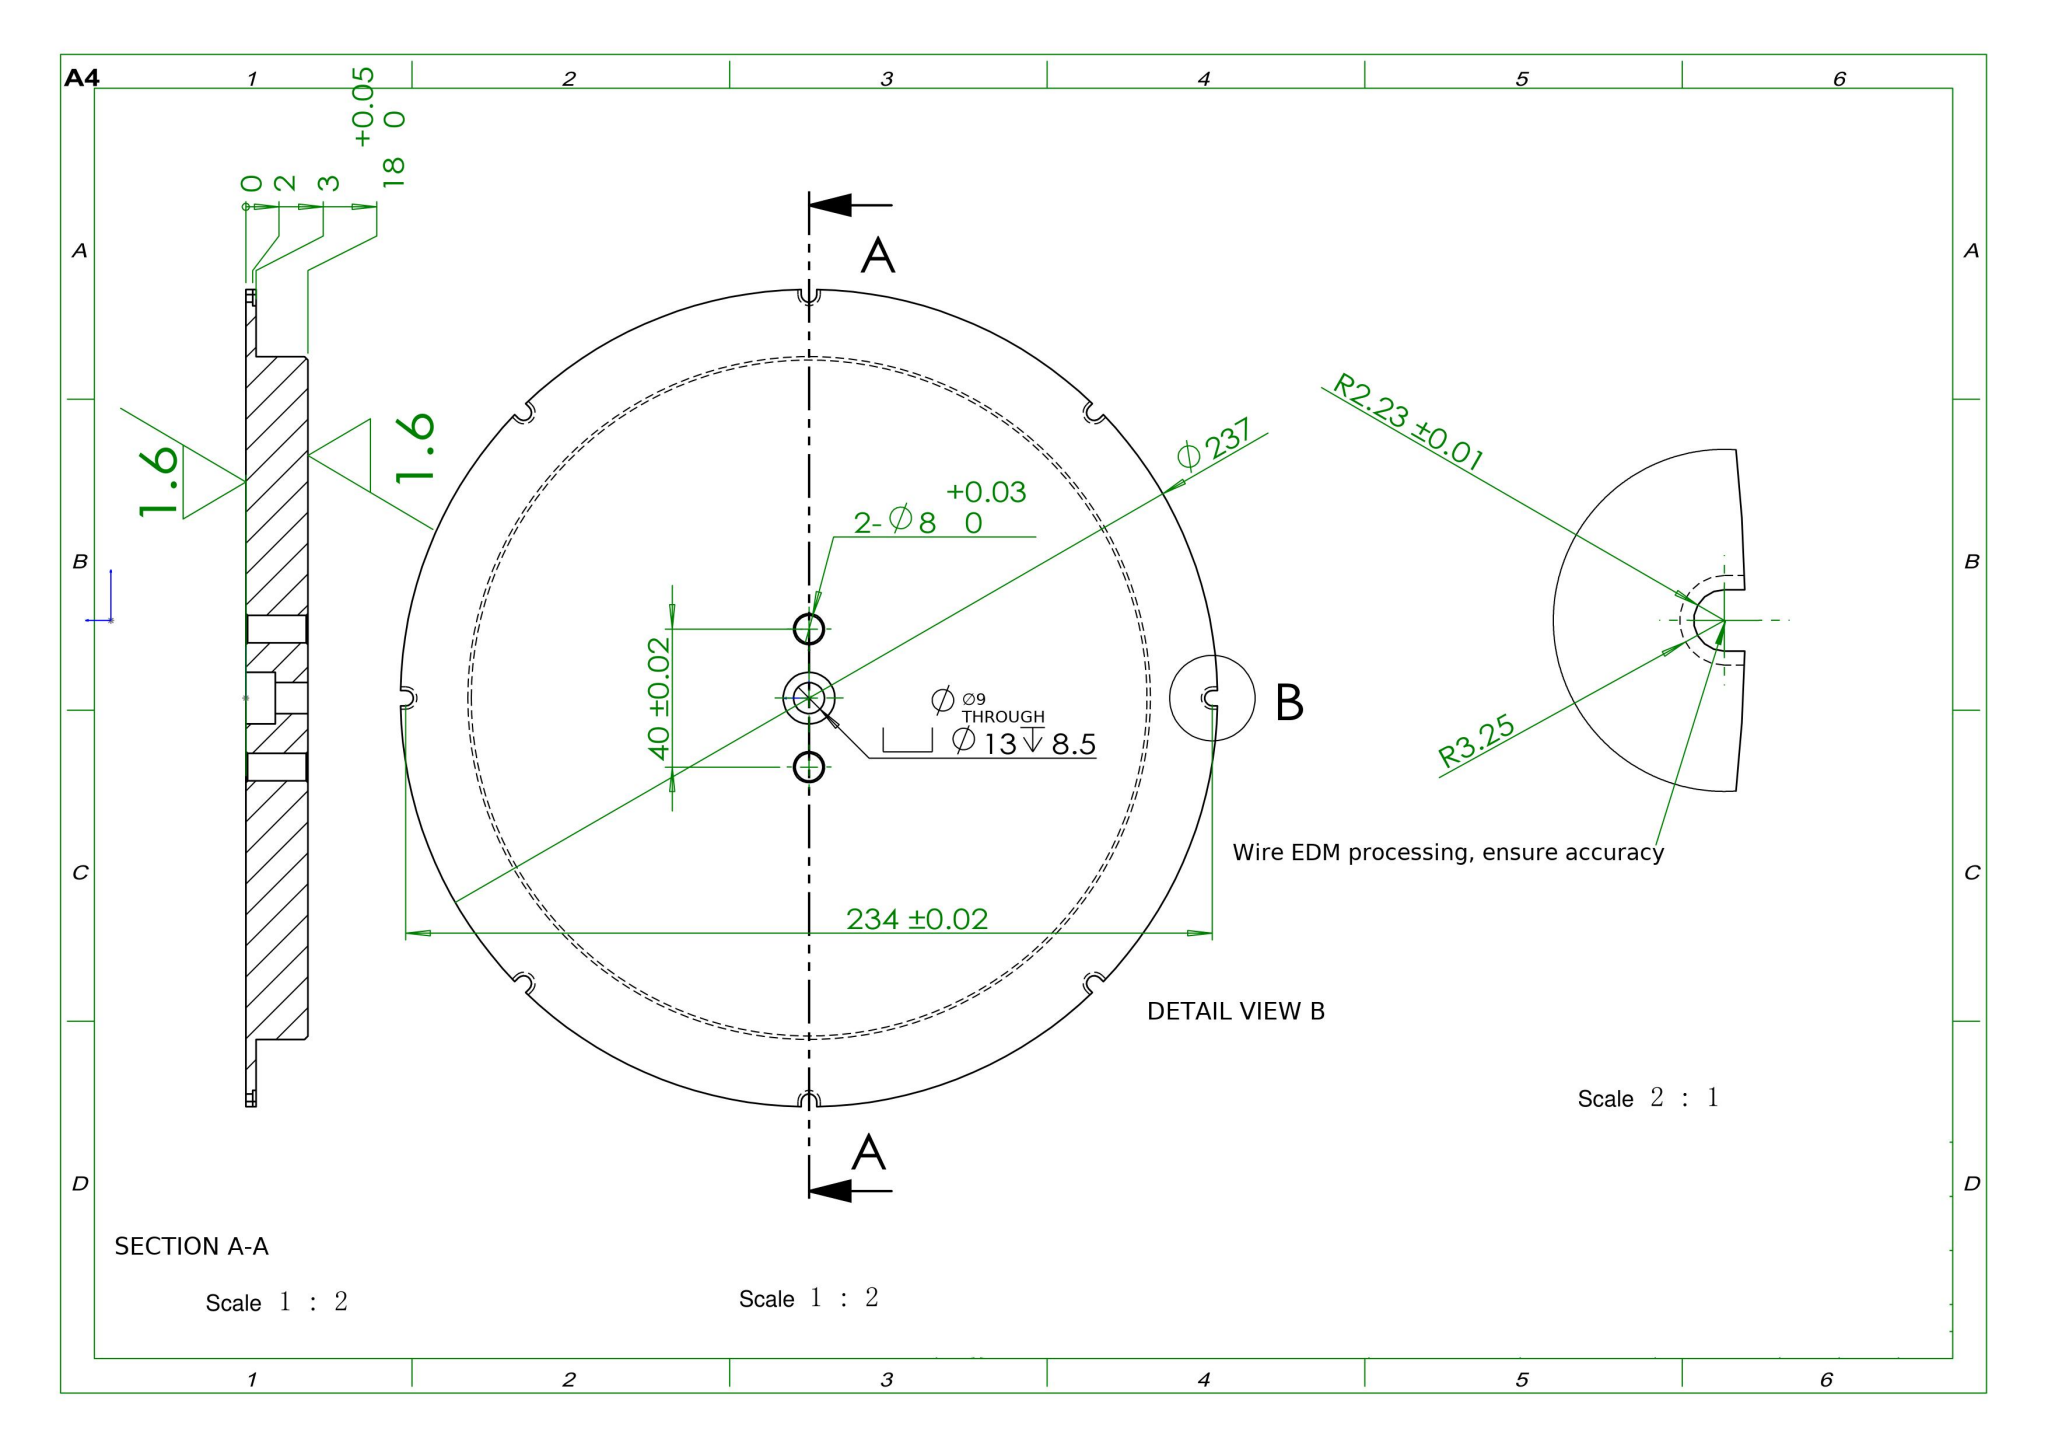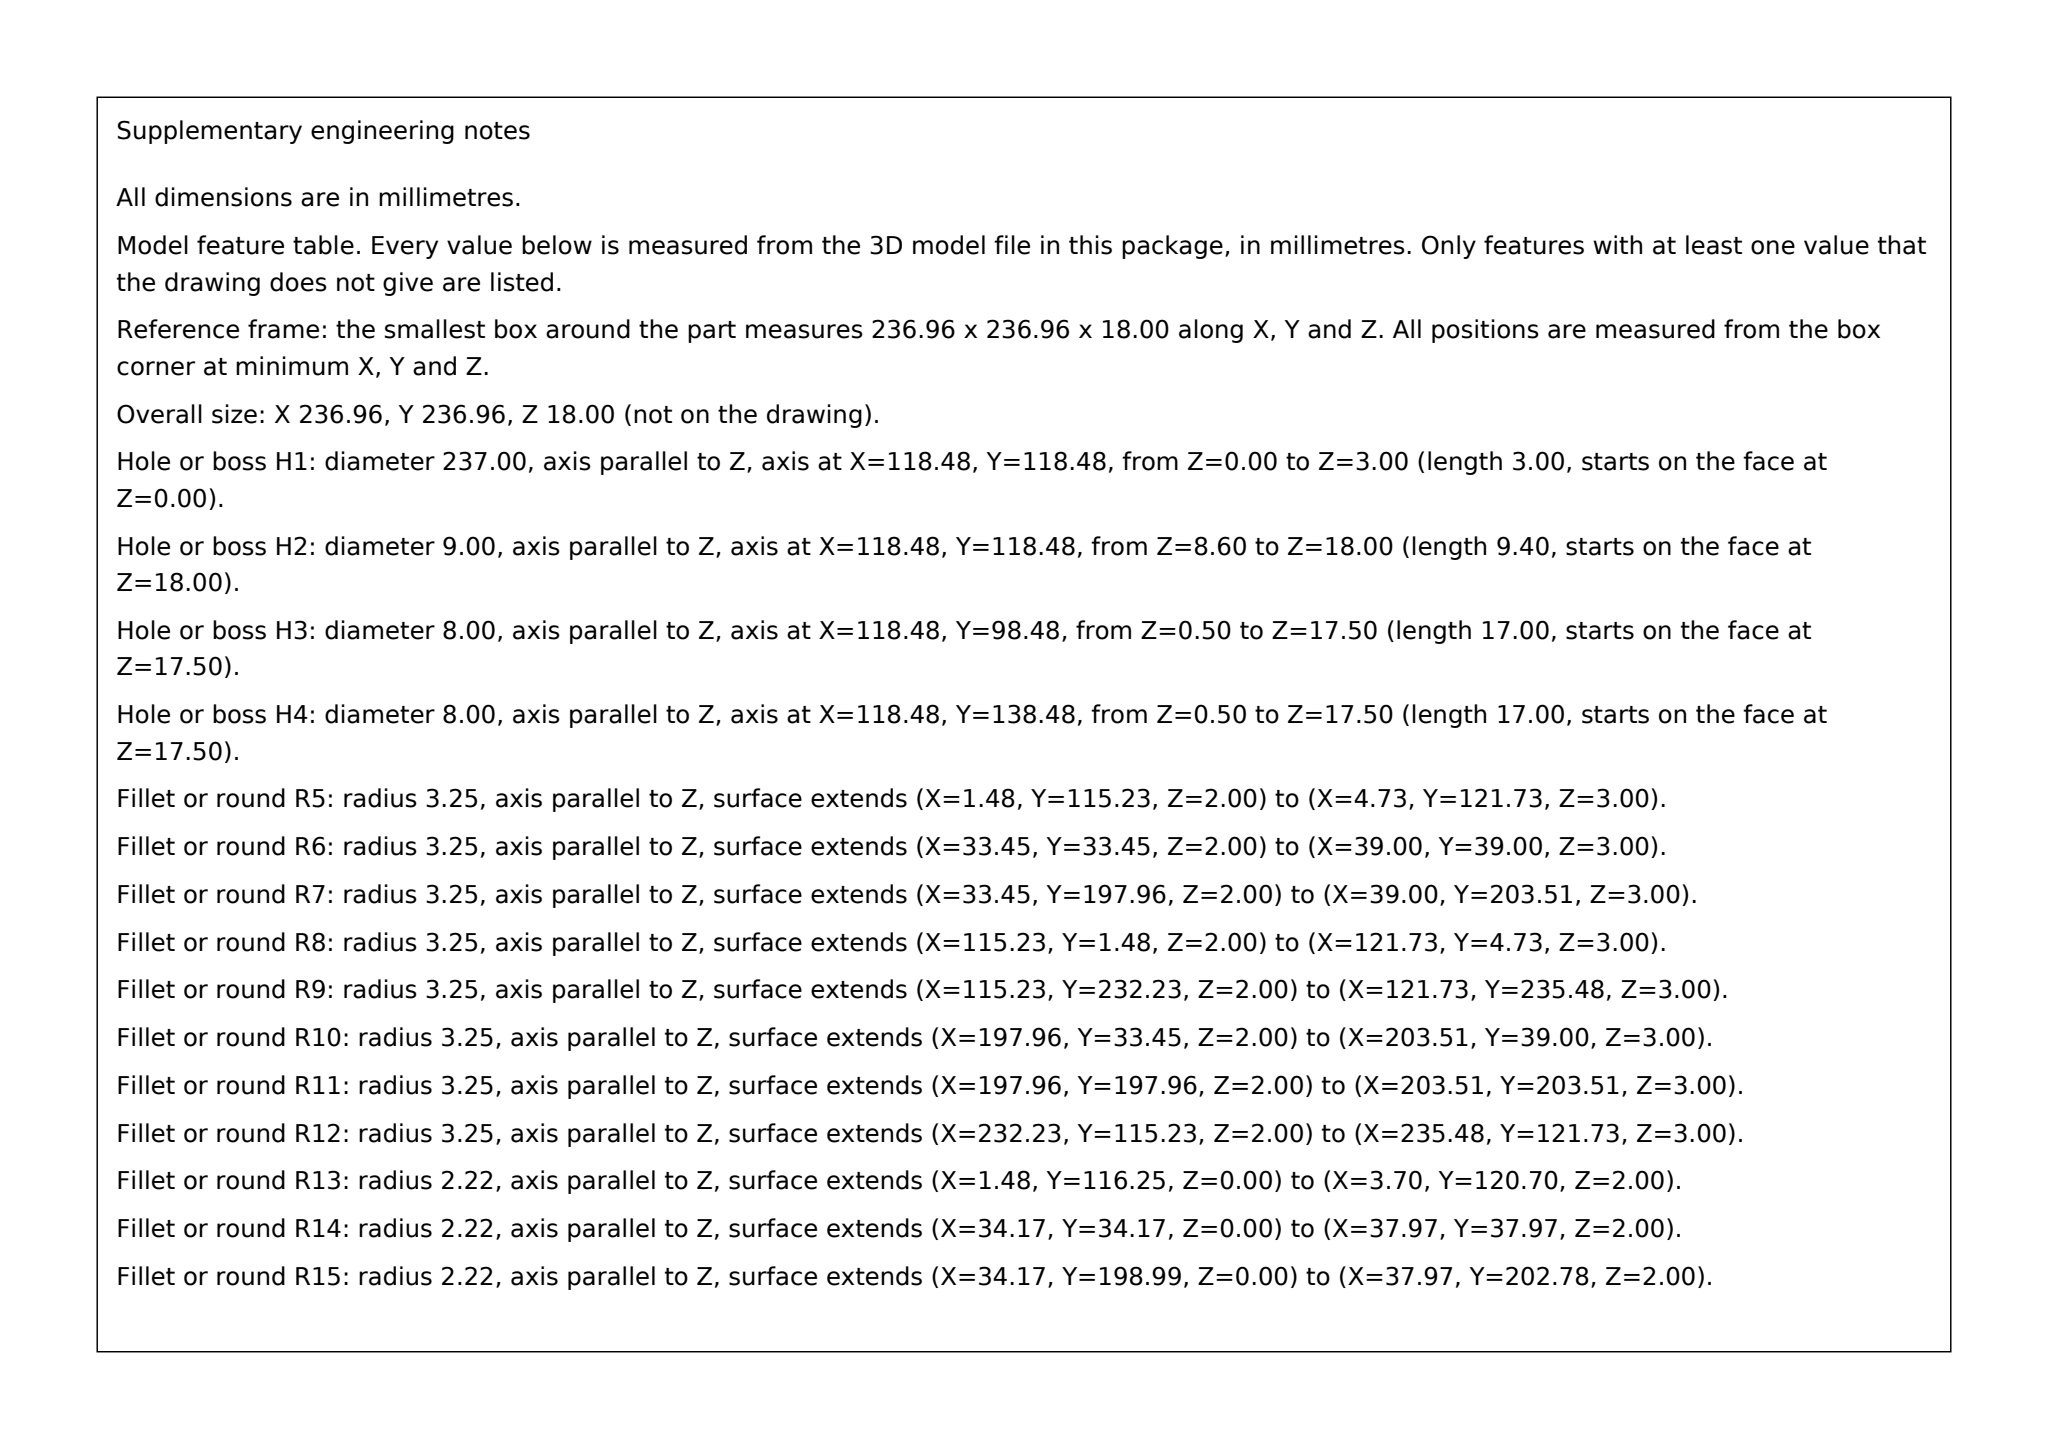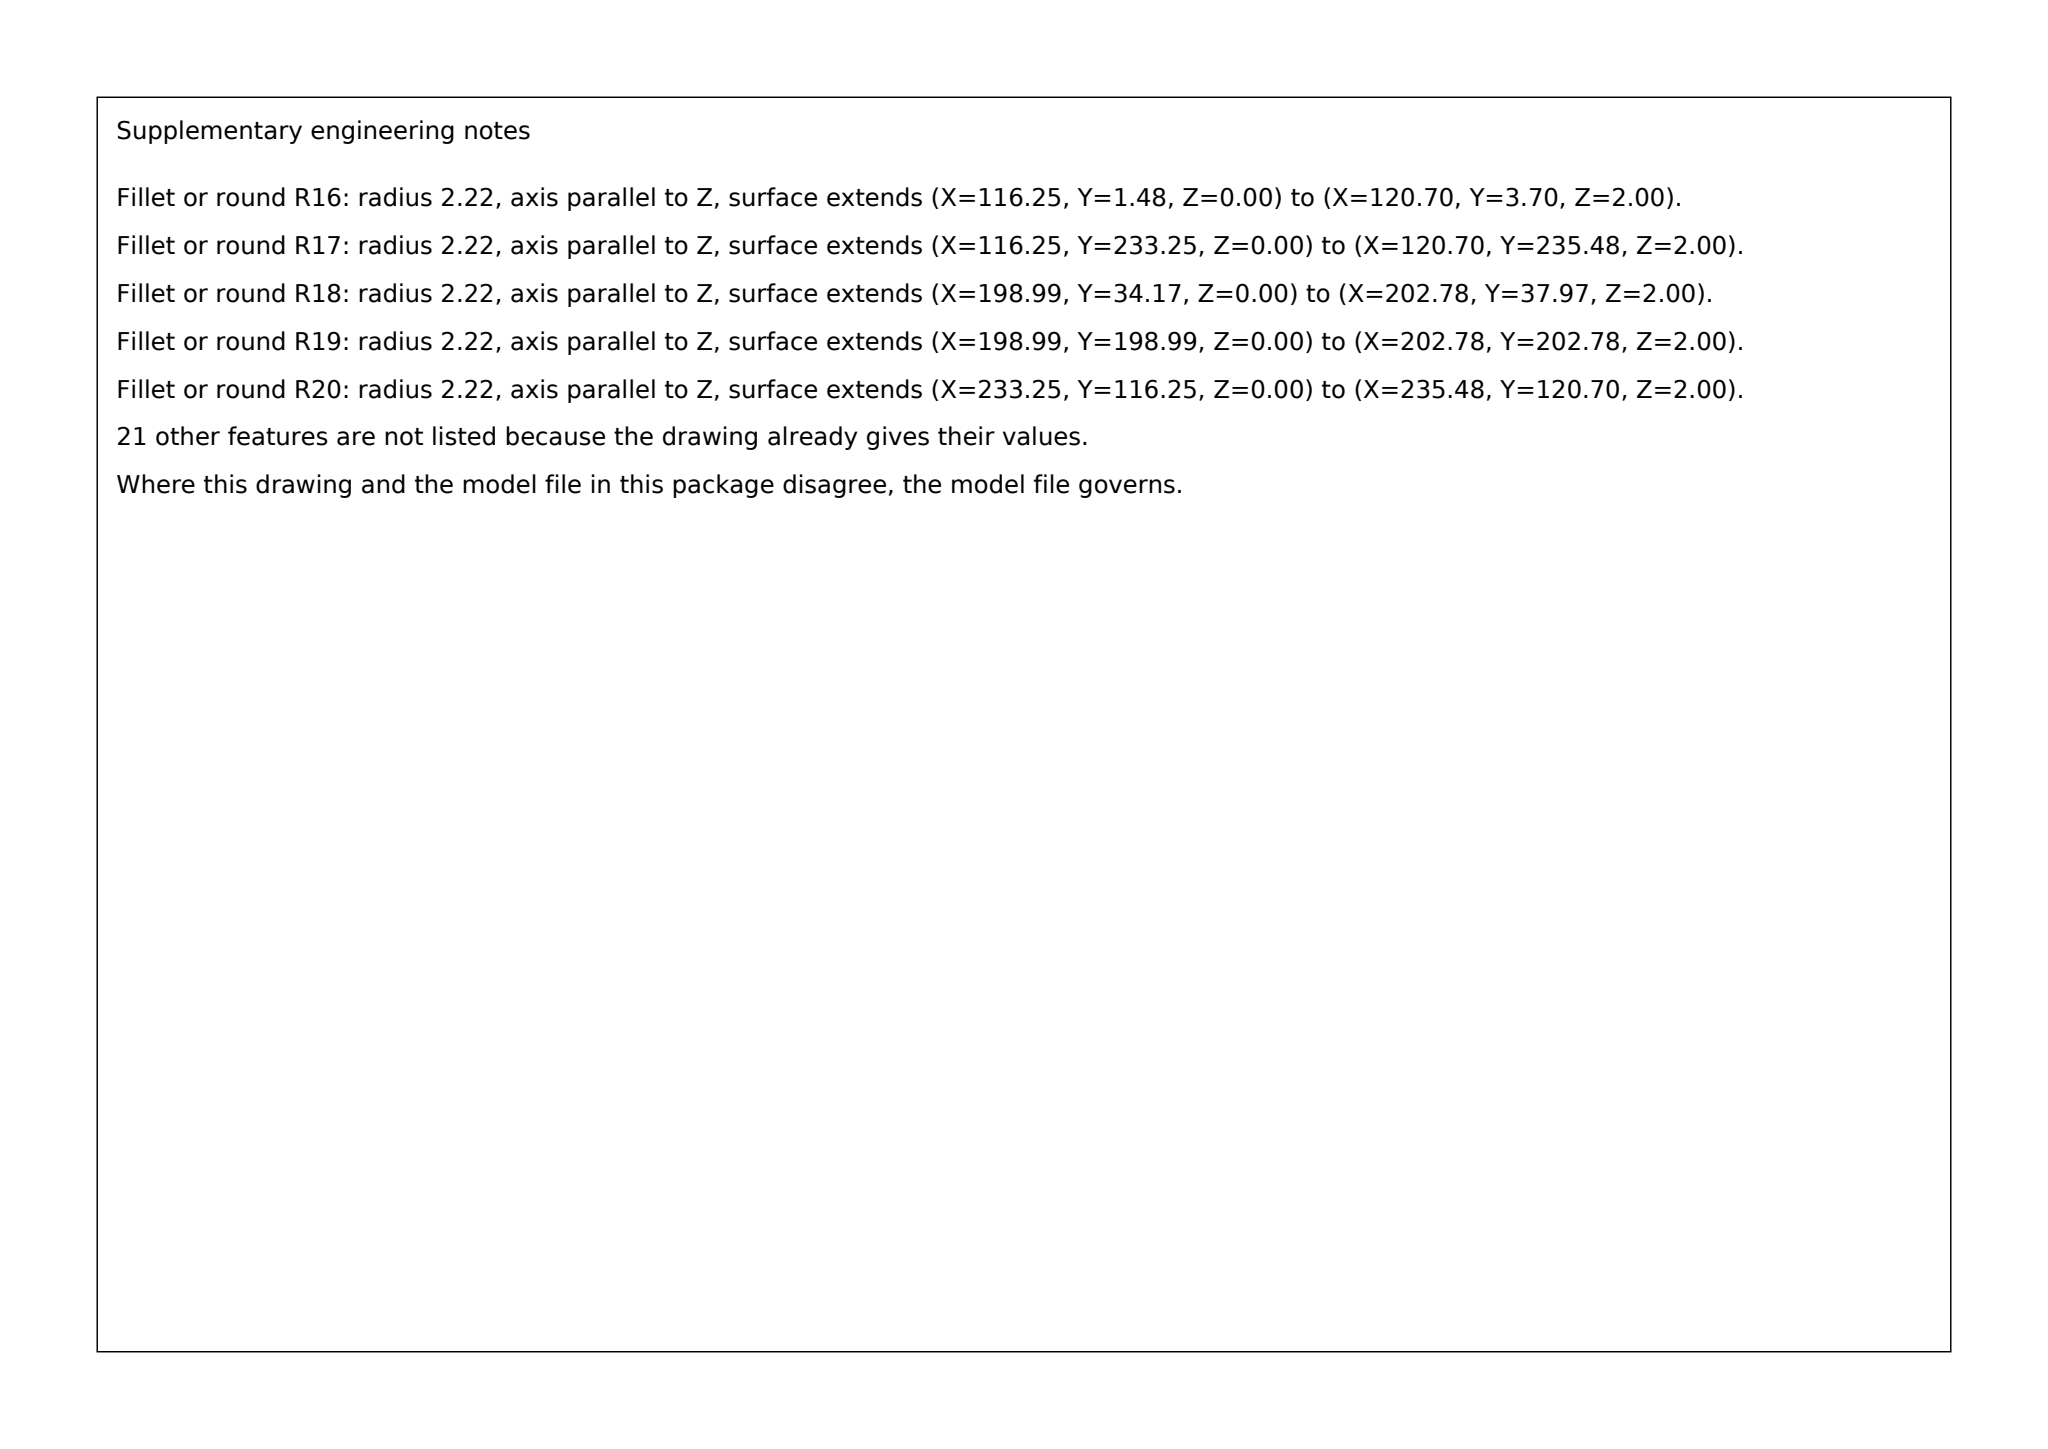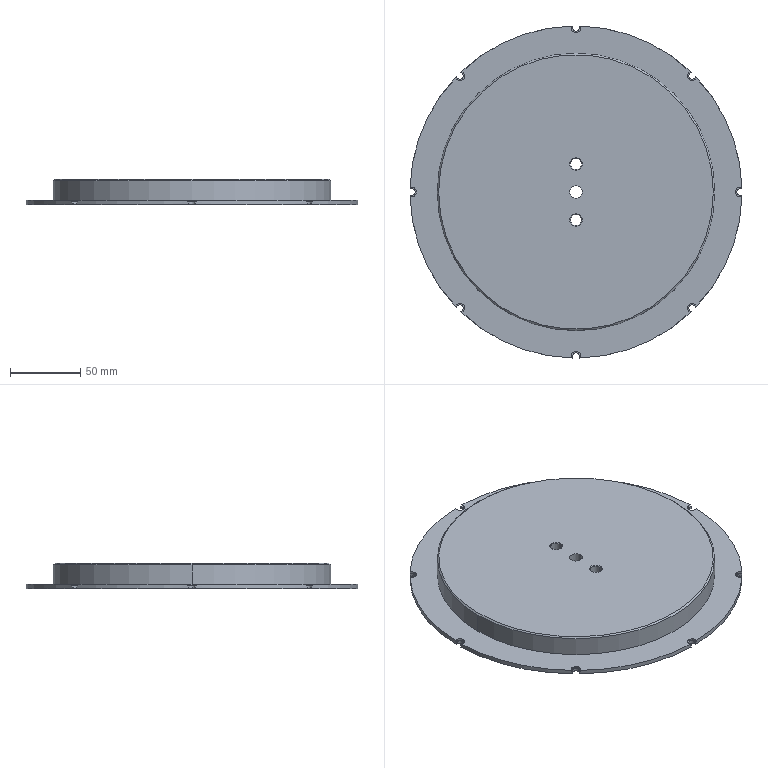Part | SolidWorks | mm | 1 solid | 94 faces | box 236.96 x 236.96 x 18 mm | volume 589515 mm3 | plane 44 | cylinder 40 | cone 10 | commonest cylinder face diameters 4.45 x11 6.5 x11 237 x8 8 x4 15 x2 9 x2 198 x2
build123d program:
from build123d import *

# Parameters (mm, degrees)
SKETCH1_R                                       = 120
BOSS_EXTRUDE1_DEPTH                             = 3
CUT_EXTRUDE1_START                              = -1
CUT_EXTRUDE1_DEPTH                              = 1
CUT_EXTRUDE2_START                              = -2
CUT_EXTRUDE2_DEPTH                              = 2
SKETCH7_R                                       = 99
BOSS_EXTRUDE4_DEPTH                             = 15
CHAMFER2_SIZE                                   = 1
SKETCH8_R                                       = 4
CUT_EXTRUDE4_DEPTH                              = 20
M8_HEX_SOCKET_HEAD_CAP_SCREW_CBORE1_D           = 9
M8_HEX_SOCKET_HEAD_CAP_SCREW_CBORE1_DEPTH       = 18
M8_HEX_SOCKET_HEAD_CAP_SCREW_CBORE1_CBORE_D     = 15
M8_HEX_SOCKET_HEAD_CAP_SCREW_CBORE1_CBORE_DEPTH = 8.6
SKETCH11_R                                      = 4
CUT_EXTRUDE5_DEPTH                              = 20
SKETCH12_R                                      = 120
SKETCH12_R_2                                    = 118.5
CUT_EXTRUDE6_DEPTH                              = 10
CHAMFER3_SIZE                                   = 0.5


with BuildPart() as part:
    # Sketch1 → Boss-Extrude1 (new body)
    with BuildSketch(Plane.XY):
        Circle(SKETCH1_R)
    extrude(amount=BOSS_EXTRUDE1_DEPTH)

    # Sketch2 → Cut-Extrude1 (cut)
    with BuildSketch(Plane.XY.offset(3).offset(CUT_EXTRUDE1_START)):
        with BuildLine():
            Line((-3.25, 117), (-3.25, 119.956))
            ThreePointArc((-3.25, 119.956), (0, 120), (3.25, 119.956))
            Line((3.25, 119.956), (3.25, 117))
            ThreePointArc((3.25, 117), (0, 113.75), (-3.25, 117))
        make_face()
        with BuildLine():
            Line((80.433, 85.03), (82.524, 87.12))
            ThreePointArc((82.524, 87.12), (84.853, 84.853), (87.12, 82.524))
            Line((87.12, 82.524), (85.03, 80.433))
            ThreePointArc((85.03, 80.433), (80.433, 80.433), (80.433, 85.03))
        make_face()
        with BuildLine():
            Line((117, 3.25), (119.956, 3.25))
            ThreePointArc((119.956, 3.25), (120, 0), (119.956, -3.25))
            Line((119.956, -3.25), (117, -3.25))
            ThreePointArc((117, -3.25), (113.75, 0), (117, 3.25))
        make_face()
        with BuildLine():
            Line((85.03, -80.433), (87.12, -82.524))
            ThreePointArc((87.12, -82.524), (84.853, -84.853), (82.524, -87.12))
            Line((82.524, -87.12), (80.433, -85.03))
            ThreePointArc((80.433, -85.03), (80.433, -80.433), (85.03, -80.433))
        make_face()
        with BuildLine():
            Line((3.25, -117), (3.25, -119.956))
            ThreePointArc((3.25, -119.956), (0, -120), (-3.25, -119.956))
            Line((-3.25, -119.956), (-3.25, -117))
            ThreePointArc((-3.25, -117), (0, -113.75), (3.25, -117))
        make_face()
        with BuildLine():
            Line((-80.433, -85.03), (-82.524, -87.12))
            ThreePointArc((-82.524, -87.12), (-84.853, -84.853), (-87.12, -82.524))
            Line((-87.12, -82.524), (-85.03, -80.433))
            ThreePointArc((-85.03, -80.433), (-80.433, -80.433), (-80.433, -85.03))
        make_face()
        with BuildLine():
            Line((-117, -3.25), (-119.956, -3.25))
            ThreePointArc((-119.956, -3.25), (-120, 0), (-119.956, 3.25))
            Line((-119.956, 3.25), (-117, 3.25))
            ThreePointArc((-117, 3.25), (-113.75, 0), (-117, -3.25))
        make_face()
        with BuildLine():
            Line((-85.03, 80.433), (-87.12, 82.524))
            ThreePointArc((-87.12, 82.524), (-84.853, 84.853), (-82.524, 87.12))
            Line((-82.524, 87.12), (-80.433, 85.03))
            ThreePointArc((-80.433, 85.03), (-80.433, 80.433), (-85.03, 80.433))
        make_face()
    extrude(amount=CUT_EXTRUDE1_DEPTH, mode=Mode.SUBTRACT)

    # Sketch3 → Cut-Extrude2 (cut)
    with BuildSketch(Plane.XY.offset(2).offset(CUT_EXTRUDE2_START)):
        with BuildLine():
            Line((-2.225, 117), (-2.225, 119.979))
            ThreePointArc((-2.225, 119.979), (0, 120), (2.225, 119.979))
            Line((2.225, 119.979), (2.225, 117))
            ThreePointArc((2.225, 117), (0, 114.775), (-2.225, 117))
        make_face()
        with BuildLine():
            Line((81.158, 84.305), (83.265, 86.412))
            ThreePointArc((83.265, 86.412), (84.853, 84.853), (86.412, 83.265))
            Line((86.412, 83.265), (84.305, 81.158))
            ThreePointArc((84.305, 81.158), (81.158, 81.158), (81.158, 84.305))
        make_face()
        with BuildLine():
            Line((117, 2.225), (119.979, 2.225))
            ThreePointArc((119.979, 2.225), (120, 0), (119.979, -2.225))
            Line((119.979, -2.225), (117, -2.225))
            ThreePointArc((117, -2.225), (114.775, 0), (117, 2.225))
        make_face()
        with BuildLine():
            Line((84.305, -81.158), (86.412, -83.265))
            ThreePointArc((86.412, -83.265), (84.853, -84.853), (83.265, -86.412))
            Line((83.265, -86.412), (81.158, -84.305))
            ThreePointArc((81.158, -84.305), (81.158, -81.158), (84.305, -81.158))
        make_face()
        with BuildLine():
            Line((2.225, -117), (2.225, -119.979))
            ThreePointArc((2.225, -119.979), (0, -120), (-2.225, -119.979))
            Line((-2.225, -119.979), (-2.225, -117))
            ThreePointArc((-2.225, -117), (0, -114.775), (2.225, -117))
        make_face()
        with BuildLine():
            Line((-81.158, -84.305), (-83.265, -86.412))
            ThreePointArc((-83.265, -86.412), (-84.853, -84.853), (-86.412, -83.265))
            Line((-86.412, -83.265), (-84.305, -81.158))
            ThreePointArc((-84.305, -81.158), (-81.158, -81.158), (-81.158, -84.305))
        make_face()
        with BuildLine():
            Line((-117, -2.225), (-119.979, -2.225))
            ThreePointArc((-119.979, -2.225), (-120, 0), (-119.979, 2.225))
            Line((-119.979, 2.225), (-117, 2.225))
            ThreePointArc((-117, 2.225), (-114.775, 0), (-117, -2.225))
        make_face()
        with BuildLine():
            Line((-84.305, 81.158), (-86.412, 83.265))
            ThreePointArc((-86.412, 83.265), (-84.853, 84.853), (-83.265, 86.412))
            Line((-83.265, 86.412), (-81.158, 84.305))
            ThreePointArc((-81.158, 84.305), (-81.158, 81.158), (-84.305, 81.158))
        make_face()
    extrude(amount=CUT_EXTRUDE2_DEPTH, mode=Mode.SUBTRACT)

    # Sketch7 → Boss-Extrude4 (add)
    with BuildSketch(Plane.XY.offset(3)):
        Circle(SKETCH7_R)
    extrude(amount=BOSS_EXTRUDE4_DEPTH)

    # Chamfer2
    chamfer2_edges = [part.edges().sort_by_distance(p)[0] for p in [
        (-99, 0, 18),
    ]]
    chamfer(chamfer2_edges, length=CHAMFER2_SIZE)

    # Sketch8 → Cut-Extrude4 (cut)
    with BuildSketch(Plane(origin=(0, 0, 0), x_dir=(-1, 0, 0), z_dir=(0, 0, -1))):
        Circle(SKETCH8_R)
    extrude(amount=-CUT_EXTRUDE4_DEPTH, mode=Mode.SUBTRACT)

    # M8 Hex Socket Head Cap Screw CBORE1
    with Locations(Plane(origin=(0, 0, 0), x_dir=(-1, 0, 0), z_dir=(0, 0, -1))):
        with Locations((0, 0)):
            CounterBoreHole(M8_HEX_SOCKET_HEAD_CAP_SCREW_CBORE1_D / 2, M8_HEX_SOCKET_HEAD_CAP_SCREW_CBORE1_CBORE_D / 2, M8_HEX_SOCKET_HEAD_CAP_SCREW_CBORE1_CBORE_DEPTH, depth=M8_HEX_SOCKET_HEAD_CAP_SCREW_CBORE1_DEPTH)

    # Sketch11 → Cut-Extrude5 (cut)
    with BuildSketch(Plane(origin=(0, 0, 0), x_dir=(-1, 0, 0), z_dir=(0, 0, -1))):
        with Locations((0, 20)):
            Circle(SKETCH11_R)
        with Locations(Location((0, -20, 0), (0, 0, 180))):
            Circle(SKETCH11_R)
    extrude(amount=-CUT_EXTRUDE5_DEPTH, mode=Mode.SUBTRACT)

    # Sketch12 → Cut-Extrude6 (cut)
    with BuildSketch(Plane(origin=(0, 0, 0), x_dir=(-1, 0, 0), z_dir=(0, 0, -1))):
        Circle(SKETCH12_R)
        Circle(SKETCH12_R_2, mode=Mode.SUBTRACT)
    extrude(amount=-CUT_EXTRUDE6_DEPTH, mode=Mode.SUBTRACT)

    # Chamfer3
    chamfer3_edges = [part.edges().sort_by_distance(p)[0] for p in [
        (4, 20, 18),
        (4, 20, 0),
        (-4, -20, 18),
        (-4, -20, 0),
    ]]
    chamfer(chamfer3_edges, length=CHAMFER3_SIZE)


solid = part.part